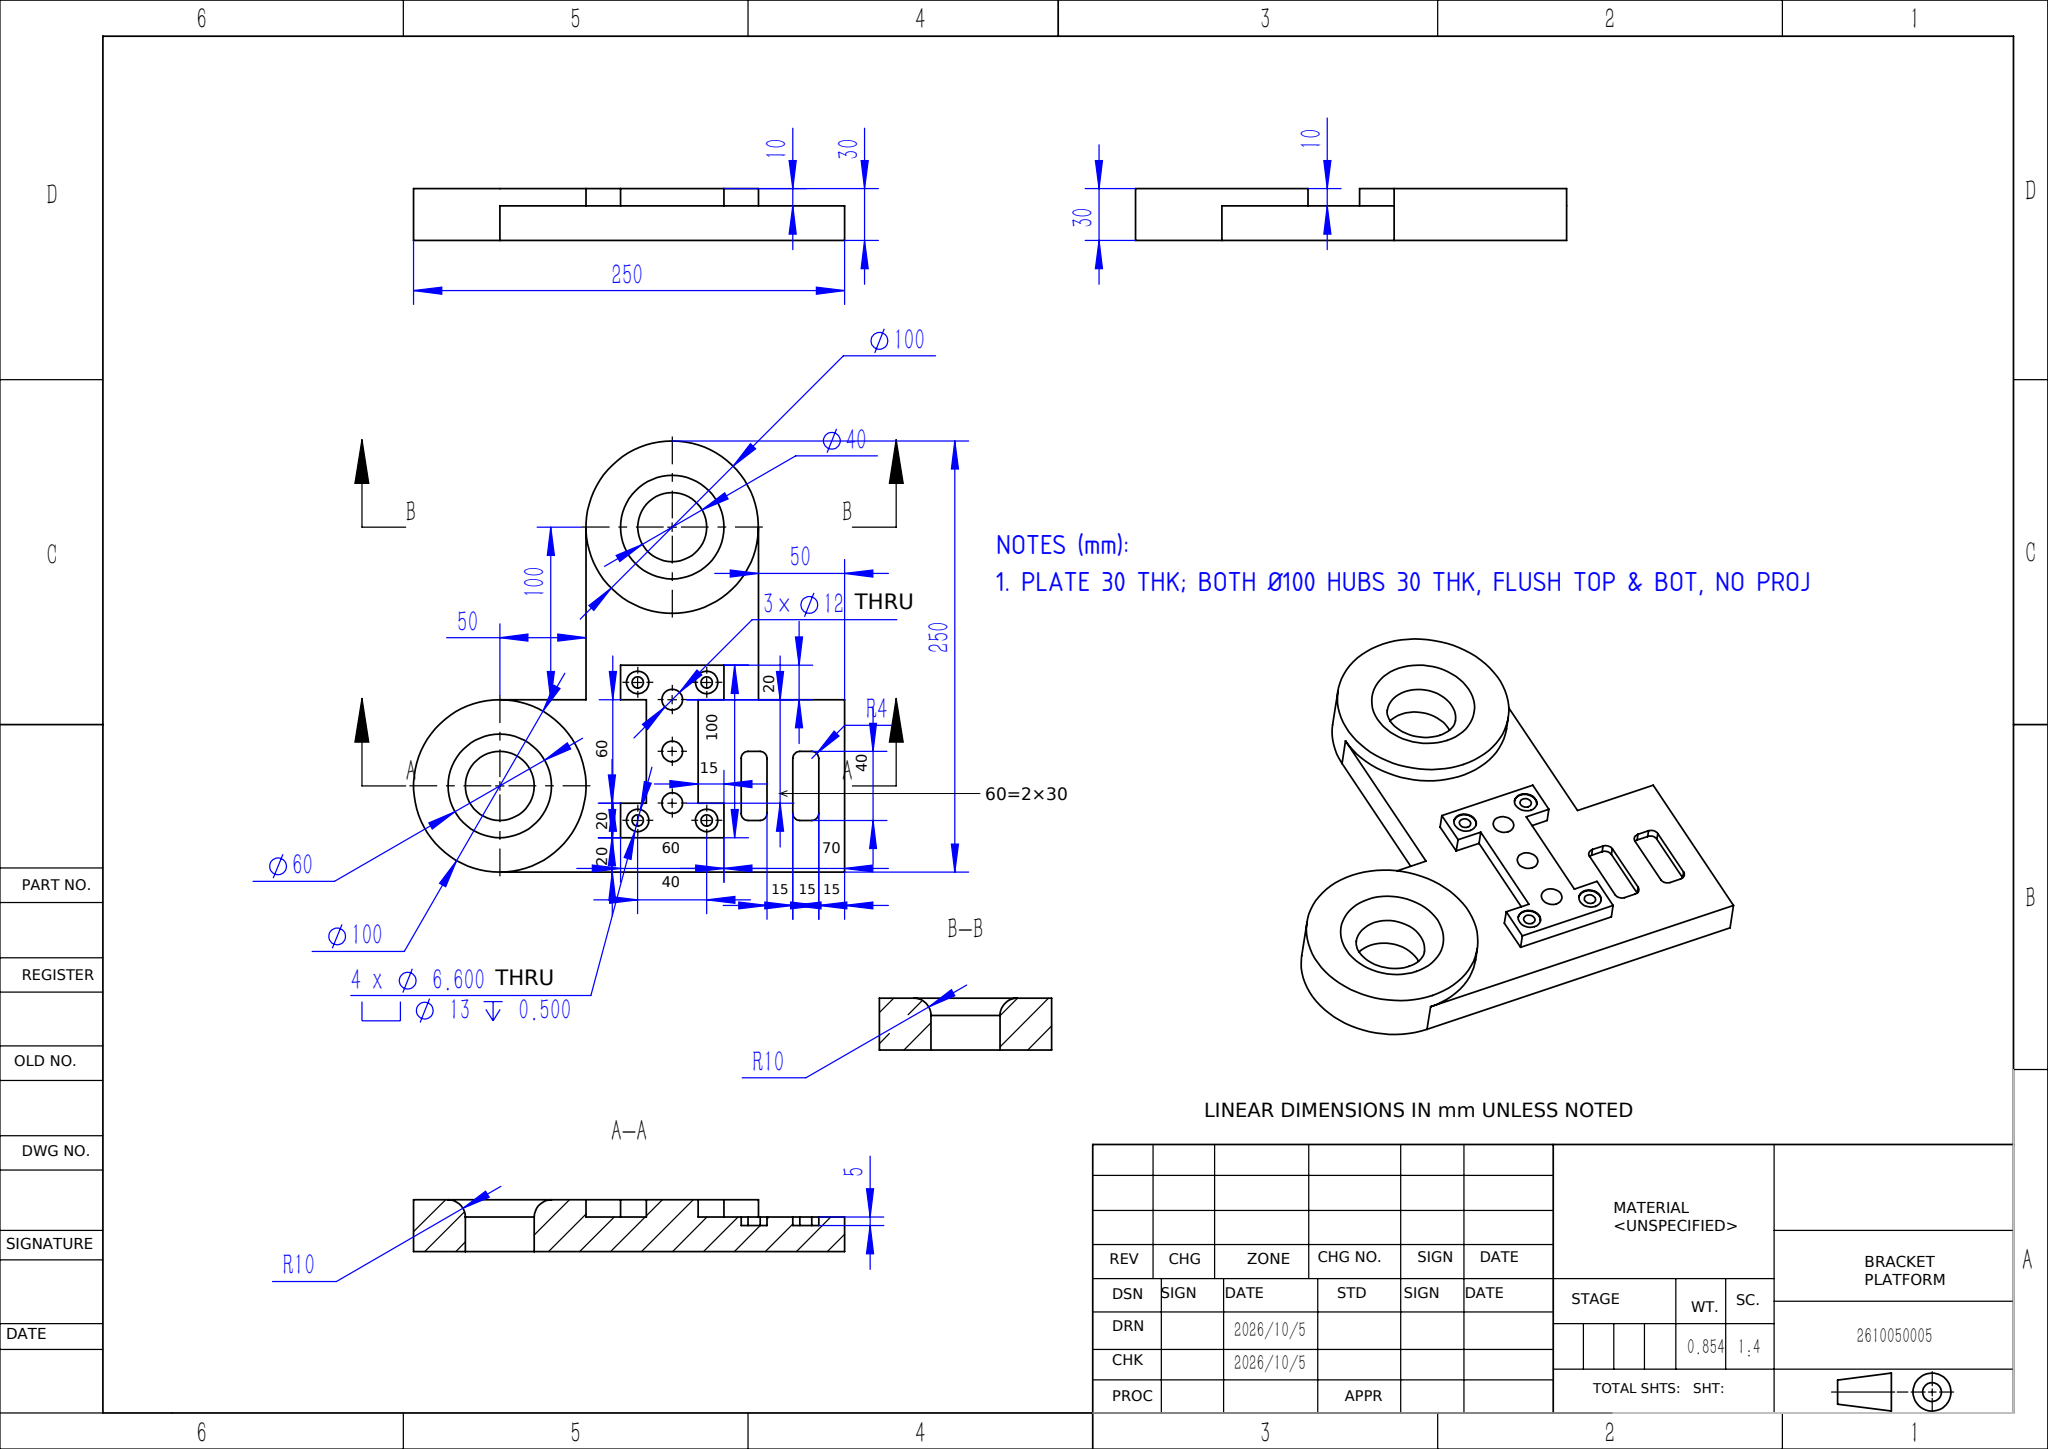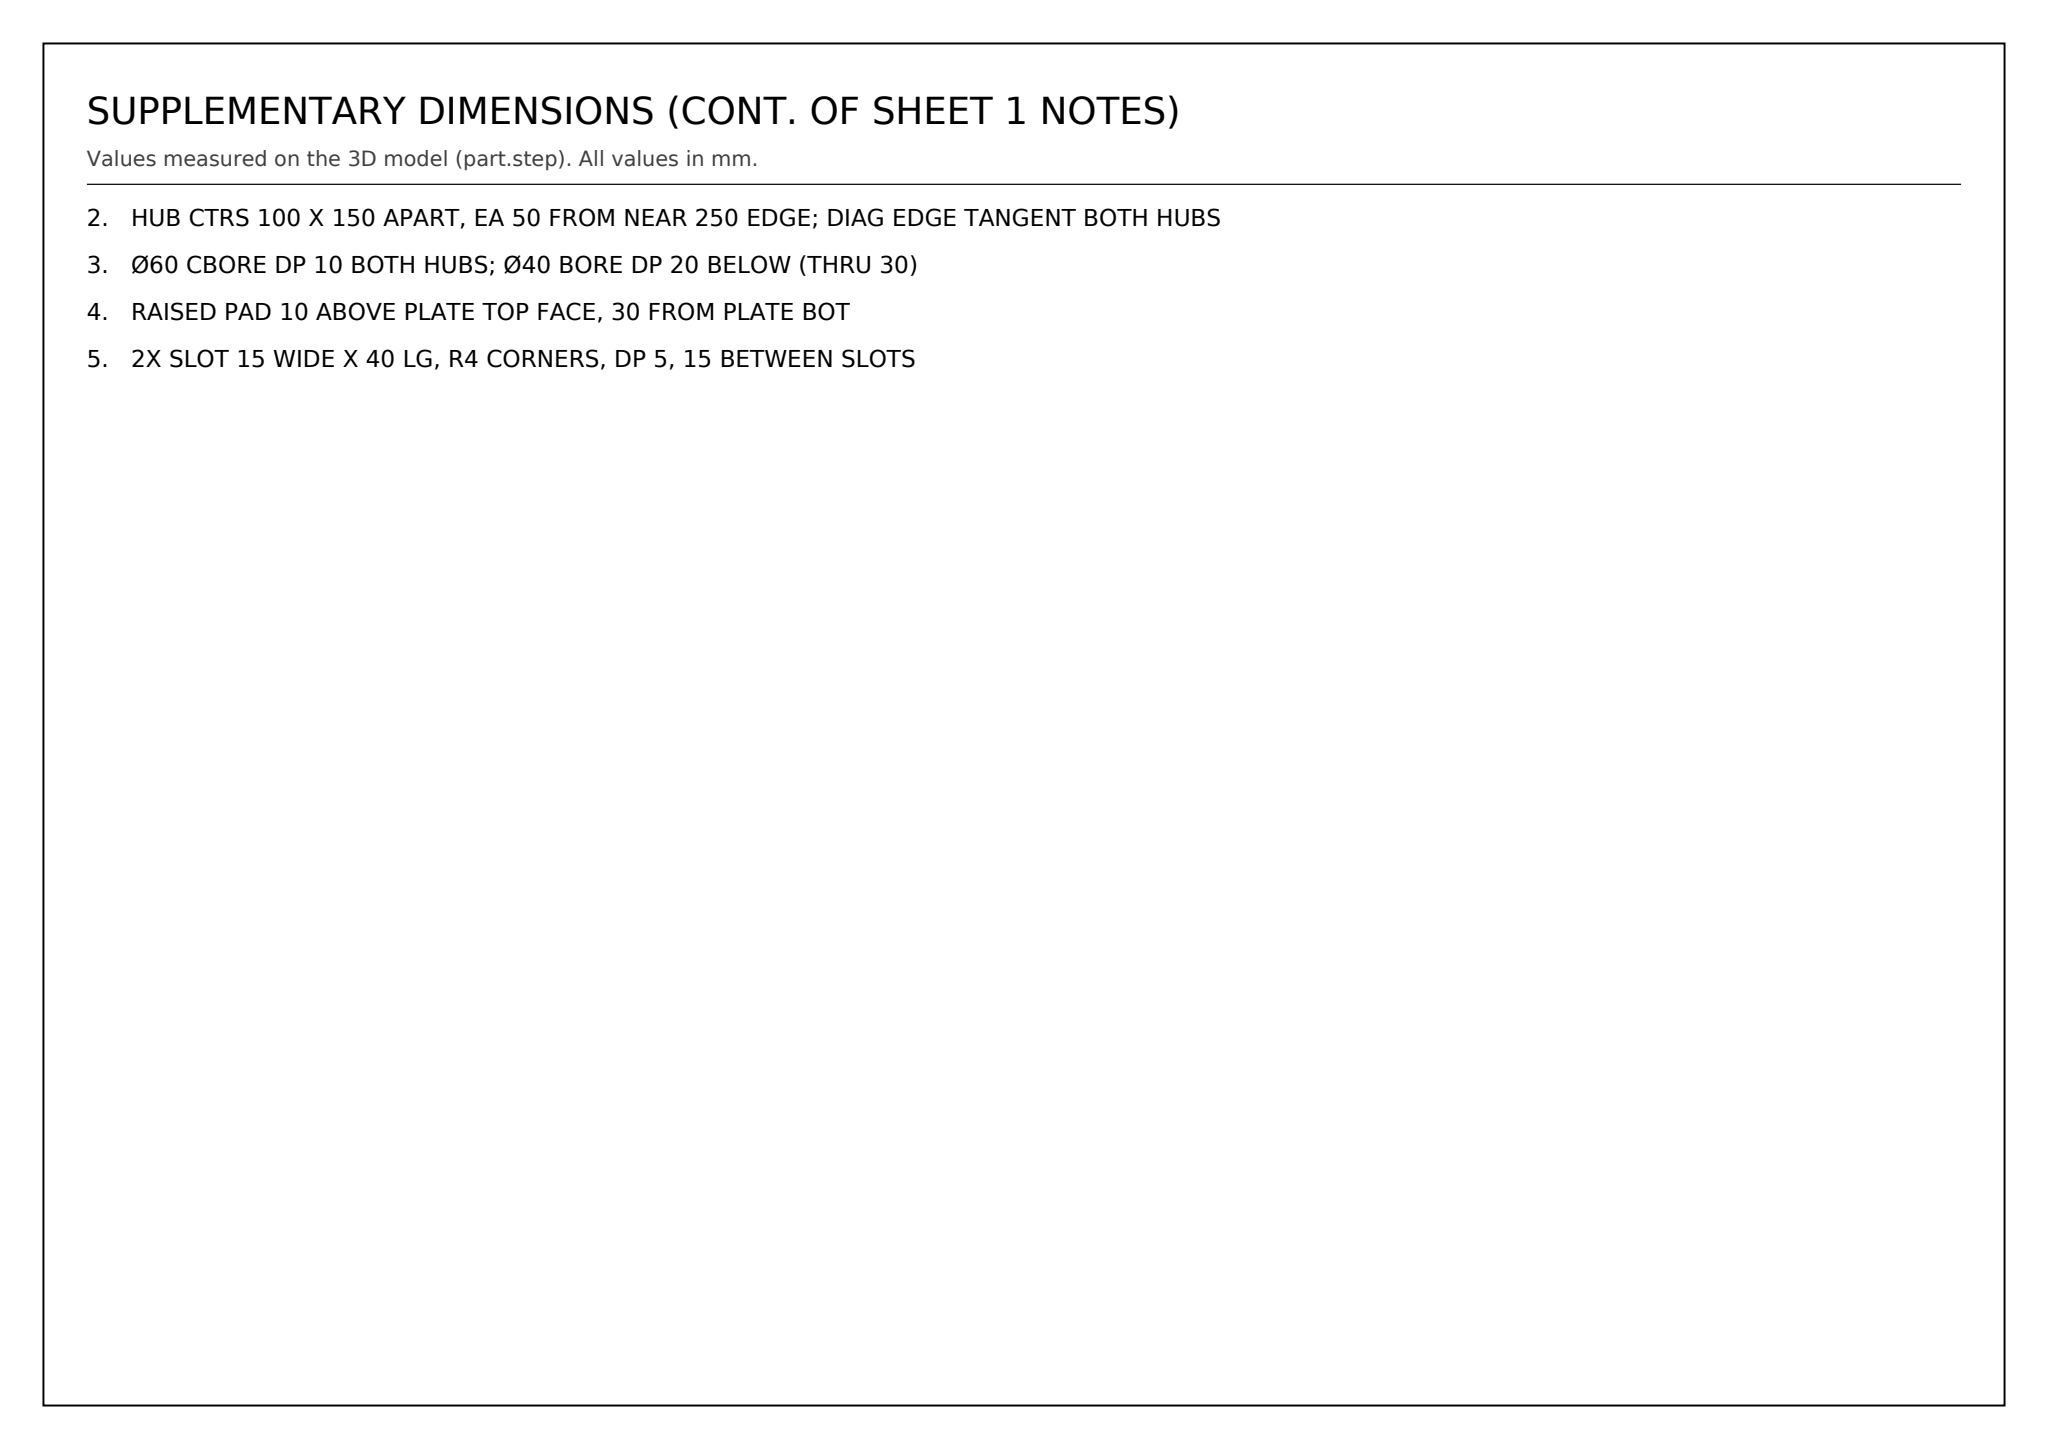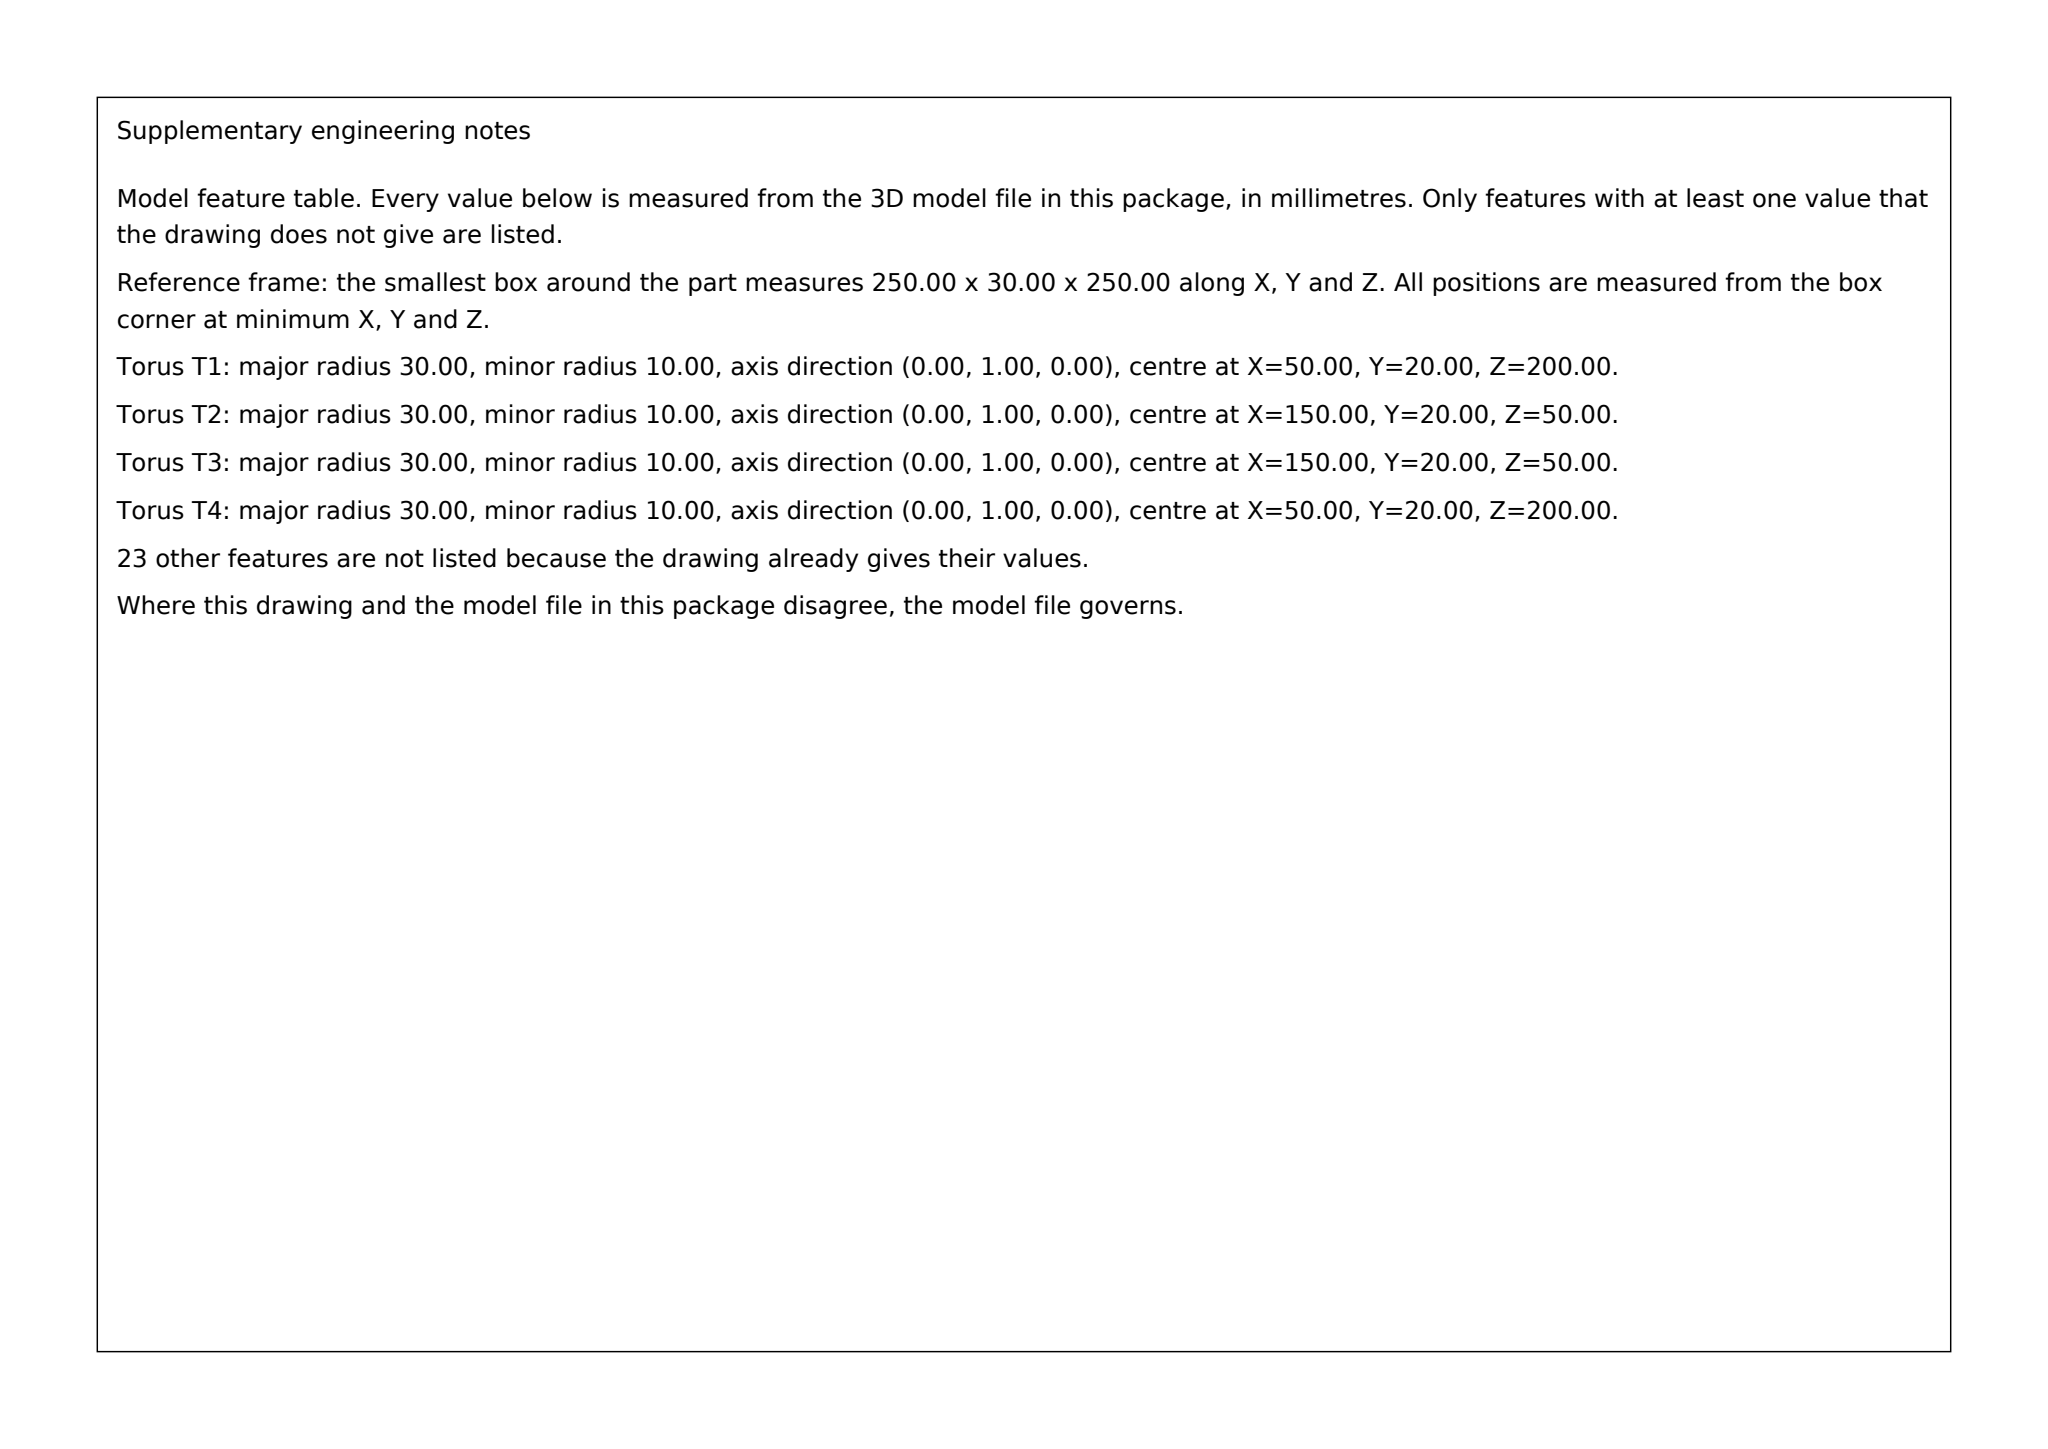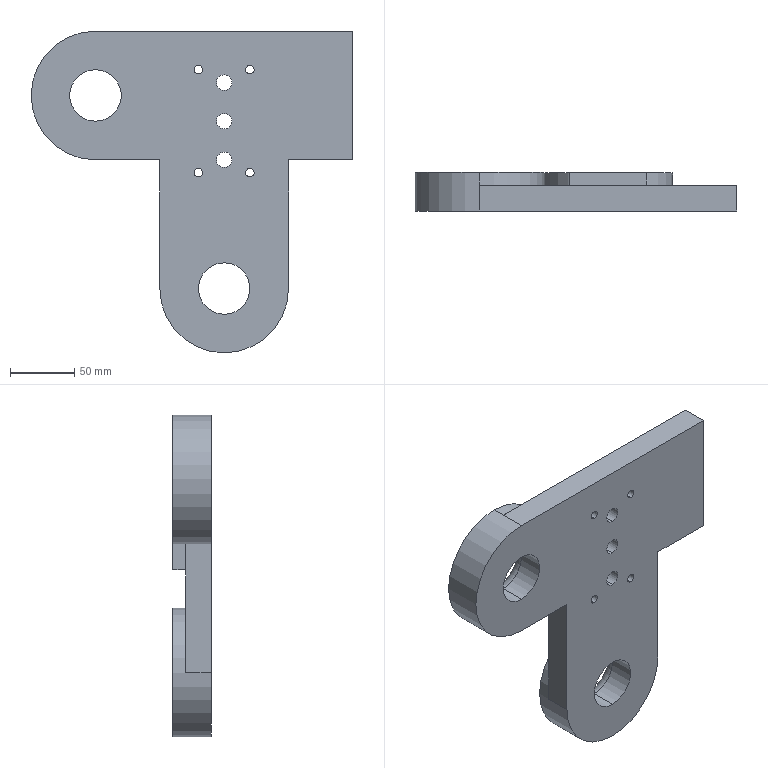Part | SolidWorks | mm | 1 solid | 79 faces | box 250 x 30 x 250 mm | volume 854421 mm3 | cylinder 38 | plane 37 | torus 4 | commonest cylinder face diameters 13 x8 6.6 x8 8 x8 12 x6 40 x4 100 x4
Drawing notes:
PLATE 30 THK; BOTH Ø100 HUBS 30 THK, FLUSH TOP & BOT, NO PROJ | from the solid: Cyl Ø100 L=30 at (50,200) and (150,50); plate y 0-30 (bbox y=30)
HUB CTRS 100 X 150 APART, EA 50 FROM NEAR 250 EDGE; DIAG EDGE TANGENT BOTH HUBS | from the solid: Hub axes x50/z200 and x150/z50: dx=100, dz=150, atan(100/150)=33.7 deg; 50 from z=0 and z=250 faces
Ø60 CBORE DP 10 BOTH HUBS; Ø40 BORE DP 20 BELOW (THRU 30) | from the solid: Ø40 bore L=20 -> 30-20=10 recess depth; Ø100 L=10 step
RAISED PAD 10 ABOVE PLATE TOP FACE, 30 FROM PLATE BOT | from the solid: y planes 20 (plate top) and 30 (pad top, = Ø6.6 CBORE 29.5+0.5); bbox y=30
2X SLOT 15 WIDE X 40 LG, R4 CORNERS, DP 5, 15 BETWEEN SLOTS | from the solid: Ø8 (R4) corner cyls L=5 at x=194/201 & 224/231, z=184/216; planes x=190,205,220,235 & z=180,220
build123d program:
from build123d import *

# Parameters (mm, degrees)
BOSS_EXTRUDE1_DEPTH                           = 10
CUT_EXTRUDE1_DEPTH                            = 5
SKETCH3_R                                     = 50
BOSS_EXTRUDE2_DEPTH                           = 10
SKETCH4_R                                     = 20
CUT_EXTRUDE2_DEPTH                            = 322.559
FILLET1_R                                     = 10
BOSS_EXTRUDE3_DEPTH                           = 10
COUNTERBORE_FOR_M6_HEX_HEAD_BOLT1_D           = 6.6
COUNTERBORE_FOR_M6_HEX_HEAD_BOLT1_CBORE_D     = 13
COUNTERBORE_FOR_M6_HEX_HEAD_BOLT1_CBORE_DEPTH = 0.5
SKETCH9_R                                     = 6
CUT_EXTRUDE3_DEPTH                            = 322.559


with BuildPart() as part:
    # Sketch1 → Boss-Extrude1 (new, symmetric)
    with BuildSketch(Plane(origin=(0, 0, 0), x_dir=(1, 0, 0), z_dir=(0, 1, 0))):
        with BuildLine():
            Line((-150, 50), (-150, 150))
            ThreePointArc((-150, 150), (-100, 200), (-50, 150))
            Line((-50, 150), (-50, 50))
            Line((-50, 50), (0, 50))
            Line((0, 50), (0, -50))
            Line((0, -50), (-200, -50))
            ThreePointArc((-200, -50), (-250, 0), (-200, 50))
            Line((-200, 50), (-150, 50))
        make_face()
    extrude(amount=BOSS_EXTRUDE1_DEPTH, both=True)

    # Sketch2 → Cut-Extrude1 (cut)
    with BuildSketch(Plane(origin=(0, 10, 0), x_dir=(1, 0, 0), z_dir=(0, 1, 0))):
        with BuildLine():
            Line((-26, 20), (-19, 20))
            ThreePointArc((-19, 20), (-16.172, 18.828), (-15, 16))
            Line((-15, 16), (-15, -16))
            ThreePointArc((-15, -16), (-16.172, -18.828), (-19, -20))
            Line((-19, -20), (-26, -20))
            ThreePointArc((-26, -20), (-28.828, -18.828), (-30, -16))
            Line((-30, -16), (-30, 16))
            ThreePointArc((-30, 16), (-28.828, 18.828), (-26, 20))
        make_face()
        with BuildLine():
            Line((-56, 20), (-49, 20))
            ThreePointArc((-49, 20), (-46.172, 18.828), (-45, 16))
            Line((-45, 16), (-45, -16))
            ThreePointArc((-45, -16), (-46.172, -18.828), (-49, -20))
            Line((-49, -20), (-56, -20))
            ThreePointArc((-56, -20), (-58.828, -18.828), (-60, -16))
            Line((-60, -16), (-60, 16))
            ThreePointArc((-60, 16), (-58.828, 18.828), (-56, 20))
        make_face()
    extrude(amount=-CUT_EXTRUDE1_DEPTH, mode=Mode.SUBTRACT)

    # Sketch3 → Boss-Extrude2 (add, symmetric)
    with BuildSketch(Plane(origin=(0, 10, 0), x_dir=(1, 0, 0), z_dir=(0, 1, 0))):
        with Locations(Location((-200, 0, 0), (0, 0, 270))):
            Circle(SKETCH3_R)
        with Locations((-100, 150)):
            Circle(SKETCH3_R)
    extrude(amount=BOSS_EXTRUDE2_DEPTH, both=True)

    # Sketch4 → Cut-Extrude2 (cut, through all)
    with BuildSketch(Plane(origin=(0, 20, 0), x_dir=(1, 0, 0), z_dir=(0, 1, 0))):
        with Locations(Location((-200, 0, 0), (0, 0, 270))):
            Circle(SKETCH4_R)
        with Locations(Location((-100, 150, 0), (0, 0, 270))):
            Circle(SKETCH4_R)
    extrude(amount=-CUT_EXTRUDE2_DEPTH, mode=Mode.SUBTRACT)

    # Fillet1
    fillet1_edges = [part.edges().sort_by_distance(p)[0] for p in [
        (-100, 20, -170),
        (-200, 20, -20),
    ]]
    fillet(fillet1_edges, radius=FILLET1_R)

    # Sketch5 → Boss-Extrude3 (add, symmetric)
    with BuildSketch(Plane(origin=(0, 10, 0), x_dir=(1, 0, 0), z_dir=(0, 1, 0))):
        Polygon((-85, -10), (-70, -10), (-70, -30), (-130, -30), (-130, -10), (-115, -10), (-115, 50), (-130, 50), (-130, 70), (-70, 70), (-70, 50), (-85, 50), align=None)
    extrude(amount=BOSS_EXTRUDE3_DEPTH, both=True)

    # Counterbore for M6 Hex Head Bolt1 (through all)
    with Locations(Plane(origin=(0, 20, 0), x_dir=(1, 0, 0), z_dir=(0, 1, 0))):
        with Locations((-120, 60), (-80, 60), (-120, -20), (-80, -20)):
            CounterBoreHole(COUNTERBORE_FOR_M6_HEX_HEAD_BOLT1_D / 2, COUNTERBORE_FOR_M6_HEX_HEAD_BOLT1_CBORE_D / 2, COUNTERBORE_FOR_M6_HEX_HEAD_BOLT1_CBORE_DEPTH)

    # Sketch9 → Cut-Extrude3 (cut, through all)
    with BuildSketch(Plane(origin=(0, 20, 0), x_dir=(1, 0, 0), z_dir=(0, 1, 0))):
        with Locations(Location((-100, 50, 0), (0, 0, 270))):
            Circle(SKETCH9_R)
        with Locations(Location((-100, 20, 0), (0, 0, 270))):
            Circle(SKETCH9_R)
        with Locations(Location((-100, -10, 0), (0, 0, 270))):
            Circle(SKETCH9_R)
    extrude(amount=-CUT_EXTRUDE3_DEPTH, mode=Mode.SUBTRACT)


solid = part.part